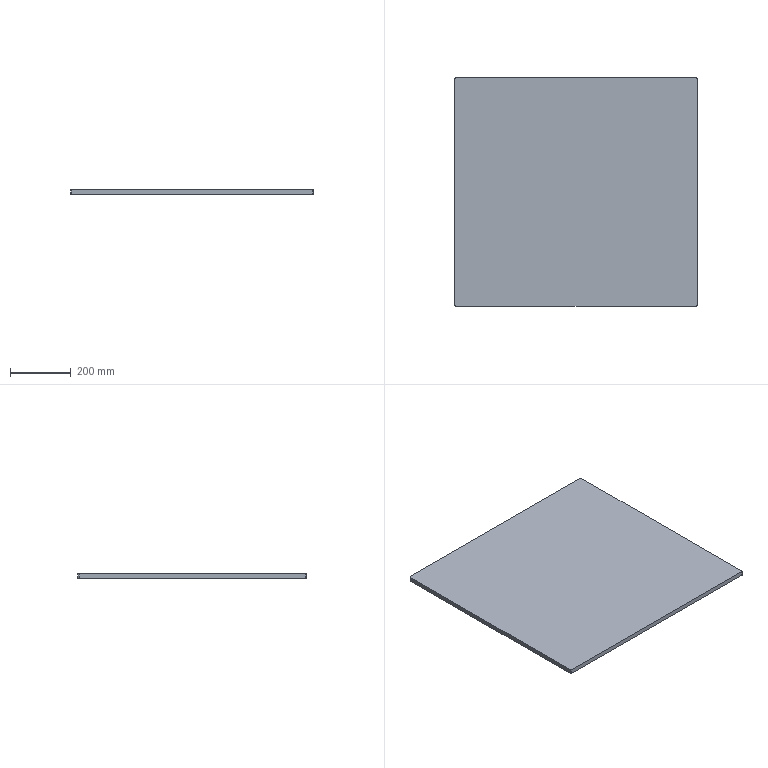Component | SolidWorks | dub02-B-1 | 1 solid | 10 faces | box 800 x 755 x 15 mm | volume 9059781 mm3 | plane 6 | cylinder 4 | commonest cylinder face diameters 6 x2 10 x2 | material Pine
build123d program:
from build123d import *

# Parameters (mm, degrees)
SKETCH1_W           = 800
SKETCH1_H           = 755
BOSS_EXTRUDE1_DEPTH = 15
FILLET2_R           = 3
FILLET3_R           = 5


with BuildPart() as part:
    # Sketch1 → Boss-Extrude1 (new body)
    with BuildSketch(Plane(origin=(0, 0, 0), x_dir=(0, 0, -1), z_dir=(1, 0, 0))):
        Rectangle(SKETCH1_W, SKETCH1_H)
    extrude(amount=BOSS_EXTRUDE1_DEPTH)

    # Fillet2
    fillet2_edges = [part.edges().sort_by_distance(p)[0] for p in [
        (7.5, -377.5, -400),
        (7.5, -377.5, 400),
    ]]
    fillet(fillet2_edges, radius=FILLET2_R)

    # Fillet3
    fillet3_edges = [part.edges().sort_by_distance(p)[0] for p in [
        (7.5, 377.5, 400),
        (7.5, 377.5, -400),
    ]]
    fillet(fillet3_edges, radius=FILLET3_R)


solid = part.part

# Placed as in the assembly
solid = solid.moved(Location((-443.006, -391.913, -1242.928), (0, 90, 0)))
STEP:
#1=COLOUR_RGB('',0.7922,0.8196,0.9333);
#2=FILL_AREA_STYLE_COLOUR('',#1);
#3=FILL_AREA_STYLE('',(#2));
#4=SURFACE_STYLE_FILL_AREA(#3);
#5=SURFACE_SIDE_STYLE('',(#4));
#6=SURFACE_STYLE_USAGE(.BOTH.,#5);
#7=PRESENTATION_STYLE_ASSIGNMENT((#6));
#8=CARTESIAN_POINT('',(-33.189,-30.174,-48.934));
#9=VERTEX_POINT('',#8);
#10=CARTESIAN_POINT('',(-33.189,-0.7643,-48.934));
#11=VERTEX_POINT('',#10);
#12=CARTESIAN_POINT('',(-33.189,-0.5674,-48.934));
#13=DIRECTION('',(-0.,1.,-0.));
#14=VECTOR('',#13,39.37);
#15=LINE('',#12,#14);
#16=EDGE_CURVE('',#9,#11,#15,.T.);
#17=ORIENTED_EDGE('',*,*,#16,.T.);
#18=CARTESIAN_POINT('',(-33.189,-0.7643,-49.525));
#19=VERTEX_POINT('',#18);
#20=CARTESIAN_POINT('',(-33.189,-0.7643,-49.525));
#21=DIRECTION('',(0.,-0.,-1.));
#22=VECTOR('',#21,39.37);
#23=LINE('',#20,#22);
#24=EDGE_CURVE('',#11,#19,#23,.T.);
#25=ORIENTED_EDGE('',*,*,#24,.T.);
#26=CARTESIAN_POINT('',(-33.189,-30.174,-49.525));
#27=VERTEX_POINT('',#26);
#28=CARTESIAN_POINT('',(-33.189,-0.5674,-49.525));
#29=DIRECTION('',(-0.,1.,-0.));
#30=VECTOR('',#29,39.37);
#31=LINE('',#28,#30);
#32=EDGE_CURVE('',#27,#19,#31,.T.);
#33=ORIENTED_EDGE('',*,*,#32,.F.);
#34=CARTESIAN_POINT('',(-33.189,-30.174,-49.525));
#35=DIRECTION('',(-0.,0.,1.));
#36=VECTOR('',#35,39.37);
#37=LINE('',#34,#36);
#38=EDGE_CURVE('',#27,#9,#37,.T.);
#39=ORIENTED_EDGE('',*,*,#38,.T.);
#40=EDGE_LOOP('',(#17,#25,#33,#39));
#41=FACE_OUTER_BOUND('',#40,.T.);
#42=CARTESIAN_POINT('',(-33.189,-0.5674,-49.525));
#43=DIRECTION('',(1.,0.,0.));
#44=DIRECTION('',(0.,-1.,0.));
#45=AXIS2_PLACEMENT_3D('',#42,#43,#44);
#46=PLANE('',#45);
#47=ADVANCED_FACE('',(#41),#46,.F.);
#48=CARTESIAN_POINT('',(-32.992,-0.5674,-48.934));
#49=VERTEX_POINT('',#48);
#50=CARTESIAN_POINT('',(-1.89,-0.5674,-48.934));
#51=VERTEX_POINT('',#50);
#52=CARTESIAN_POINT('',(-1.693,-0.5674,-48.934));
#53=DIRECTION('',(1.,0.,0.));
#54=VECTOR('',#53,39.37);
#55=LINE('',#52,#54);
#56=EDGE_CURVE('',#49,#51,#55,.T.);
#57=ORIENTED_EDGE('',*,*,#56,.T.);
#58=CARTESIAN_POINT('',(-1.89,-0.5674,-49.525));
#59=VERTEX_POINT('',#58);
#60=CARTESIAN_POINT('',(-1.89,-0.5674,-49.525));
#61=DIRECTION('',(0.,-0.,-1.));
#62=VECTOR('',#61,39.37);
#63=LINE('',#60,#62);
#64=EDGE_CURVE('',#51,#59,#63,.T.);
#65=ORIENTED_EDGE('',*,*,#64,.T.);
#66=CARTESIAN_POINT('',(-32.992,-0.5674,-49.525));
#67=VERTEX_POINT('',#66);
#68=CARTESIAN_POINT('',(-1.693,-0.5674,-49.525));
#69=DIRECTION('',(1.,0.,0.));
#70=VECTOR('',#69,39.37);
#71=LINE('',#68,#70);
#72=EDGE_CURVE('',#67,#59,#71,.T.);
#73=ORIENTED_EDGE('',*,*,#72,.F.);
#74=CARTESIAN_POINT('',(-32.992,-0.5674,-49.525));
#75=DIRECTION('',(-0.,0.,1.));
#76=VECTOR('',#75,39.37);
#77=LINE('',#74,#76);
#78=EDGE_CURVE('',#67,#49,#77,.T.);
#79=ORIENTED_EDGE('',*,*,#78,.T.);
#80=EDGE_LOOP('',(#57,#65,#73,#79));
#81=FACE_OUTER_BOUND('',#80,.T.);
#82=CARTESIAN_POINT('',(-1.693,-0.5674,-49.525));
#83=DIRECTION('',(0.,-1.,0.));
#84=DIRECTION('',(-1.,-0.,-0.));
#85=AXIS2_PLACEMENT_3D('',#82,#83,#84);
#86=PLANE('',#85);
#87=ADVANCED_FACE('',(#81),#86,.F.);
#88=CARTESIAN_POINT('',(-1.693,-0.7643,-49.525));
#89=VERTEX_POINT('',#88);
#90=CARTESIAN_POINT('',(-1.693,-30.174,-49.525));
#91=VERTEX_POINT('',#90);
#92=CARTESIAN_POINT('',(-1.693,-0.5674,-49.525));
#93=DIRECTION('',(0.,-1.,0.));
#94=VECTOR('',#93,39.37);
#95=LINE('',#92,#94);
#96=EDGE_CURVE('',#89,#91,#95,.T.);
#97=ORIENTED_EDGE('',*,*,#96,.F.);
#98=CARTESIAN_POINT('',(-1.693,-0.7643,-48.934));
#99=VERTEX_POINT('',#98);
#100=CARTESIAN_POINT('',(-1.693,-0.7643,-49.525));
#101=DIRECTION('',(-0.,0.,1.));
#102=VECTOR('',#101,39.37);
#103=LINE('',#100,#102);
#104=EDGE_CURVE('',#89,#99,#103,.T.);
#105=ORIENTED_EDGE('',*,*,#104,.T.);
#106=CARTESIAN_POINT('',(-1.693,-30.174,-48.934));
#107=VERTEX_POINT('',#106);
#108=CARTESIAN_POINT('',(-1.693,-0.5674,-48.934));
#109=DIRECTION('',(0.,-1.,0.));
#110=VECTOR('',#109,39.37);
#111=LINE('',#108,#110);
#112=EDGE_CURVE('',#99,#107,#111,.T.);
#113=ORIENTED_EDGE('',*,*,#112,.T.);
#114=CARTESIAN_POINT('',(-1.693,-30.174,-49.525));
#115=DIRECTION('',(0.,-0.,-1.));
#116=VECTOR('',#115,39.37);
#117=LINE('',#114,#116);
#118=EDGE_CURVE('',#107,#91,#117,.T.);
#119=ORIENTED_EDGE('',*,*,#118,.T.);
#120=EDGE_LOOP('',(#97,#105,#113,#119));
#121=FACE_OUTER_BOUND('',#120,.T.);
#122=CARTESIAN_POINT('',(-1.693,-0.5674,-49.525));
#123=DIRECTION('',(-1.,-0.,-0.));
#124=DIRECTION('',(-0.,1.,-0.));
#125=AXIS2_PLACEMENT_3D('',#122,#123,#124);
#126=PLANE('',#125);
#127=ADVANCED_FACE('',(#121),#126,.F.);
#128=CARTESIAN_POINT('',(-1.811,-30.292,-48.934));
#129=VERTEX_POINT('',#128);
#130=CARTESIAN_POINT('',(-33.071,-30.292,-48.934));
#131=VERTEX_POINT('',#130);
#132=CARTESIAN_POINT('',(-1.693,-30.292,-48.934));
#133=DIRECTION('',(-1.,-0.,-0.));
#134=VECTOR('',#133,39.37);
#135=LINE('',#132,#134);
#136=EDGE_CURVE('',#129,#131,#135,.T.);
#137=ORIENTED_EDGE('',*,*,#136,.T.);
#138=CARTESIAN_POINT('',(-33.071,-30.292,-49.525));
#139=VERTEX_POINT('',#138);
#140=CARTESIAN_POINT('',(-33.071,-30.292,-49.525));
#141=DIRECTION('',(0.,-0.,-1.));
#142=VECTOR('',#141,39.37);
#143=LINE('',#140,#142);
#144=EDGE_CURVE('',#131,#139,#143,.T.);
#145=ORIENTED_EDGE('',*,*,#144,.T.);
#146=CARTESIAN_POINT('',(-1.811,-30.292,-49.525));
#147=VERTEX_POINT('',#146);
#148=CARTESIAN_POINT('',(-1.693,-30.292,-49.525));
#149=DIRECTION('',(-1.,-0.,-0.));
#150=VECTOR('',#149,39.37);
#151=LINE('',#148,#150);
#152=EDGE_CURVE('',#147,#139,#151,.T.);
#153=ORIENTED_EDGE('',*,*,#152,.F.);
#154=CARTESIAN_POINT('',(-1.811,-30.292,-49.525));
#155=DIRECTION('',(-0.,0.,1.));
#156=VECTOR('',#155,39.37);
#157=LINE('',#154,#156);
#158=EDGE_CURVE('',#147,#129,#157,.T.);
#159=ORIENTED_EDGE('',*,*,#158,.T.);
#160=EDGE_LOOP('',(#137,#145,#153,#159));
#161=FACE_OUTER_BOUND('',#160,.T.);
#162=CARTESIAN_POINT('',(-1.693,-30.292,-49.525));
#163=DIRECTION('',(-0.,1.,-0.));
#164=DIRECTION('',(1.,0.,0.));
#165=AXIS2_PLACEMENT_3D('',#162,#163,#164);
#166=PLANE('',#165);
#167=ADVANCED_FACE('',(#161),#166,.F.);
#168=ORIENTED_EDGE('',*,*,#72,.T.);
#169=CARTESIAN_POINT('',(-1.89,-0.7643,-49.525));
#170=DIRECTION('',(0.,-0.,-1.));
#171=DIRECTION('',(-1.,0.,0.));
#172=AXIS2_PLACEMENT_3D('',#169,#170,#171);
#173=CIRCLE('',#172,0.1969);
#174=EDGE_CURVE('',#59,#89,#173,.T.);
#175=ORIENTED_EDGE('',*,*,#174,.T.);
#176=ORIENTED_EDGE('',*,*,#96,.T.);
#177=CARTESIAN_POINT('',(-1.811,-30.174,-49.525));
#178=DIRECTION('',(0.,-0.,-1.));
#179=DIRECTION('',(-1.,0.,0.));
#180=AXIS2_PLACEMENT_3D('',#177,#178,#179);
#181=CIRCLE('',#180,0.1181);
#182=EDGE_CURVE('',#91,#147,#181,.T.);
#183=ORIENTED_EDGE('',*,*,#182,.T.);
#184=ORIENTED_EDGE('',*,*,#152,.T.);
#185=CARTESIAN_POINT('',(-33.071,-30.174,-49.525));
#186=DIRECTION('',(0.,-0.,-1.));
#187=DIRECTION('',(-1.,0.,0.));
#188=AXIS2_PLACEMENT_3D('',#185,#186,#187);
#189=CIRCLE('',#188,0.1181);
#190=EDGE_CURVE('',#139,#27,#189,.T.);
#191=ORIENTED_EDGE('',*,*,#190,.T.);
#192=ORIENTED_EDGE('',*,*,#32,.T.);
#193=CARTESIAN_POINT('',(-32.992,-0.7643,-49.525));
#194=DIRECTION('',(0.,-0.,-1.));
#195=DIRECTION('',(-1.,0.,0.));
#196=AXIS2_PLACEMENT_3D('',#193,#194,#195);
#197=CIRCLE('',#196,0.1969);
#198=EDGE_CURVE('',#19,#67,#197,.T.);
#199=ORIENTED_EDGE('',*,*,#198,.T.);
#200=EDGE_LOOP('',(#168,#175,#176,#183,#184,#191,#192,#199));
#201=FACE_OUTER_BOUND('',#200,.T.);
#202=CARTESIAN_POINT('',(-17.441,-15.43,-49.525));
#203=DIRECTION('',(0.,-0.,-1.));
#204=DIRECTION('',(-1.,-0.,-0.));
#205=AXIS2_PLACEMENT_3D('',#202,#203,#204);
#206=PLANE('',#205);
#207=ADVANCED_FACE('',(#201),#206,.T.);
#208=ORIENTED_EDGE('',*,*,#112,.F.);
#209=CARTESIAN_POINT('',(-1.89,-0.7643,-48.934));
#210=DIRECTION('',(-0.,0.,1.));
#211=DIRECTION('',(-1.,0.,0.));
#212=AXIS2_PLACEMENT_3D('',#209,#210,#211);
#213=CIRCLE('',#212,0.1969);
#214=EDGE_CURVE('',#99,#51,#213,.T.);
#215=ORIENTED_EDGE('',*,*,#214,.T.);
#216=ORIENTED_EDGE('',*,*,#56,.F.);
#217=CARTESIAN_POINT('',(-32.992,-0.7643,-48.934));
#218=DIRECTION('',(-0.,0.,1.));
#219=DIRECTION('',(-1.,0.,0.));
#220=AXIS2_PLACEMENT_3D('',#217,#218,#219);
#221=CIRCLE('',#220,0.1969);
#222=EDGE_CURVE('',#49,#11,#221,.T.);
#223=ORIENTED_EDGE('',*,*,#222,.T.);
#224=ORIENTED_EDGE('',*,*,#16,.F.);
#225=CARTESIAN_POINT('',(-33.071,-30.174,-48.934));
#226=DIRECTION('',(-0.,0.,1.));
#227=DIRECTION('',(-1.,0.,0.));
#228=AXIS2_PLACEMENT_3D('',#225,#226,#227);
#229=CIRCLE('',#228,0.1181);
#230=EDGE_CURVE('',#9,#131,#229,.T.);
#231=ORIENTED_EDGE('',*,*,#230,.T.);
#232=ORIENTED_EDGE('',*,*,#136,.F.);
#233=CARTESIAN_POINT('',(-1.811,-30.174,-48.934));
#234=DIRECTION('',(-0.,0.,1.));
#235=DIRECTION('',(-1.,0.,0.));
#236=AXIS2_PLACEMENT_3D('',#233,#234,#235);
#237=CIRCLE('',#236,0.1181);
#238=EDGE_CURVE('',#129,#107,#237,.T.);
#239=ORIENTED_EDGE('',*,*,#238,.T.);
#240=EDGE_LOOP('',(#208,#215,#216,#223,#224,#231,#232,#239));
#241=FACE_OUTER_BOUND('',#240,.T.);
#242=CARTESIAN_POINT('',(-17.441,-15.43,-48.934));
#243=DIRECTION('',(0.,-0.,-1.));
#244=DIRECTION('',(-1.,-0.,-0.));
#245=AXIS2_PLACEMENT_3D('',#242,#243,#244);
#246=PLANE('',#245);
#247=ADVANCED_FACE('',(#241),#246,.F.);
#248=ORIENTED_EDGE('',*,*,#190,.F.);
#249=ORIENTED_EDGE('',*,*,#144,.F.);
#250=ORIENTED_EDGE('',*,*,#230,.F.);
#251=ORIENTED_EDGE('',*,*,#38,.F.);
#252=EDGE_LOOP('',(#248,#249,#250,#251));
#253=FACE_OUTER_BOUND('',#252,.T.);
#254=CARTESIAN_POINT('',(-33.071,-30.174,-49.525));
#255=DIRECTION('',(-0.,0.,1.));
#256=DIRECTION('',(1.,0.,0.));
#257=AXIS2_PLACEMENT_3D('',#254,#255,#256);
#258=CYLINDRICAL_SURFACE('',#257,0.1181);
#259=ADVANCED_FACE('',(#253),#258,.T.);
#260=ORIENTED_EDGE('',*,*,#182,.F.);
#261=ORIENTED_EDGE('',*,*,#118,.F.);
#262=ORIENTED_EDGE('',*,*,#238,.F.);
#263=ORIENTED_EDGE('',*,*,#158,.F.);
#264=EDGE_LOOP('',(#260,#261,#262,#263));
#265=FACE_OUTER_BOUND('',#264,.T.);
#266=CARTESIAN_POINT('',(-1.811,-30.174,-49.525));
#267=DIRECTION('',(-0.,0.,1.));
#268=DIRECTION('',(1.,0.,0.));
#269=AXIS2_PLACEMENT_3D('',#266,#267,#268);
#270=CYLINDRICAL_SURFACE('',#269,0.1181);
#271=ADVANCED_FACE('',(#265),#270,.T.);
#272=ORIENTED_EDGE('',*,*,#174,.F.);
#273=ORIENTED_EDGE('',*,*,#64,.F.);
#274=ORIENTED_EDGE('',*,*,#214,.F.);
#275=ORIENTED_EDGE('',*,*,#104,.F.);
#276=EDGE_LOOP('',(#272,#273,#274,#275));
#277=FACE_OUTER_BOUND('',#276,.T.);
#278=CARTESIAN_POINT('',(-1.89,-0.7643,-49.525));
#279=DIRECTION('',(-0.,0.,1.));
#280=DIRECTION('',(1.,0.,0.));
#281=AXIS2_PLACEMENT_3D('',#278,#279,#280);
#282=CYLINDRICAL_SURFACE('',#281,0.1969);
#283=ADVANCED_FACE('',(#277),#282,.T.);
#284=ORIENTED_EDGE('',*,*,#198,.F.);
#285=ORIENTED_EDGE('',*,*,#24,.F.);
#286=ORIENTED_EDGE('',*,*,#222,.F.);
#287=ORIENTED_EDGE('',*,*,#78,.F.);
#288=EDGE_LOOP('',(#284,#285,#286,#287));
#289=FACE_OUTER_BOUND('',#288,.T.);
#290=CARTESIAN_POINT('',(-32.992,-0.7643,-49.525));
#291=DIRECTION('',(-0.,0.,1.));
#292=DIRECTION('',(1.,0.,0.));
#293=AXIS2_PLACEMENT_3D('',#290,#291,#292);
#294=CYLINDRICAL_SURFACE('',#293,0.1969);
#295=ADVANCED_FACE('',(#289),#294,.T.);
#296=CLOSED_SHELL('',(#47,#87,#127,#167,#207,#247,#259,#271,#283,#295));
#297=MANIFOLD_SOLID_BREP('',#296);
#298=STYLED_ITEM('',(#7),#297);
#299=(LENGTH_UNIT()NAMED_UNIT(*)SI_UNIT($,.METRE.));
#300=LENGTH_MEASURE_WITH_UNIT(LENGTH_MEASURE(0.0254),#299);
#301=DIMENSIONAL_EXPONENTS(1.,0.,0.,0.,0.,0.,0.);
#302=(CONVERSION_BASED_UNIT('',#300)LENGTH_UNIT()NAMED_UNIT(#301));
#303=UNCERTAINTY_MEASURE_WITH_UNIT(LENGTH_MEASURE(0.00001),#302,'','');
#304=(NAMED_UNIT(*)PLANE_ANGLE_UNIT()SI_UNIT($,.RADIAN.));
#305=(NAMED_UNIT(*)SI_UNIT($,.STERADIAN.)SOLID_ANGLE_UNIT());
#306=(GEOMETRIC_REPRESENTATION_CONTEXT(3)GLOBAL_UNCERTAINTY_ASSIGNED_CONTEXT((#303))GLOBAL_UNIT_ASSIGNED_CONTEXT((#302,#304,#305))REPRESENTATION_CONTEXT('',''));
#307=MECHANICAL_DESIGN_GEOMETRIC_PRESENTATION_REPRESENTATION('',(#298),#306);
#308=CARTESIAN_POINT('',(0.,0.,0.));
#309=DIRECTION('',(0.,0.,1.));
#310=DIRECTION('',(1.,0.,0.));
#311=AXIS2_PLACEMENT_3D('',#308,#309,#310);
#312=(LENGTH_UNIT()NAMED_UNIT(*)SI_UNIT($,.METRE.));
#313=LENGTH_MEASURE_WITH_UNIT(LENGTH_MEASURE(0.0254),#312);
#314=DIMENSIONAL_EXPONENTS(1.,0.,0.,0.,0.,0.,0.);
#315=(CONVERSION_BASED_UNIT('',#313)LENGTH_UNIT()NAMED_UNIT(#314));
#316=UNCERTAINTY_MEASURE_WITH_UNIT(LENGTH_MEASURE(0.00001),#315,'','');
#317=(NAMED_UNIT(*)PLANE_ANGLE_UNIT()SI_UNIT($,.RADIAN.));
#318=(NAMED_UNIT(*)SI_UNIT($,.STERADIAN.)SOLID_ANGLE_UNIT());
#319=(GEOMETRIC_REPRESENTATION_CONTEXT(3)GLOBAL_UNCERTAINTY_ASSIGNED_CONTEXT((#316))GLOBAL_UNIT_ASSIGNED_CONTEXT((#315,#317,#318))REPRESENTATION_CONTEXT('',''));
#320=ADVANCED_BREP_SHAPE_REPRESENTATION('',(#297,#311),#319);
#321=PRESENTATION_LAYER_ASSIGNMENT('','',(#298));